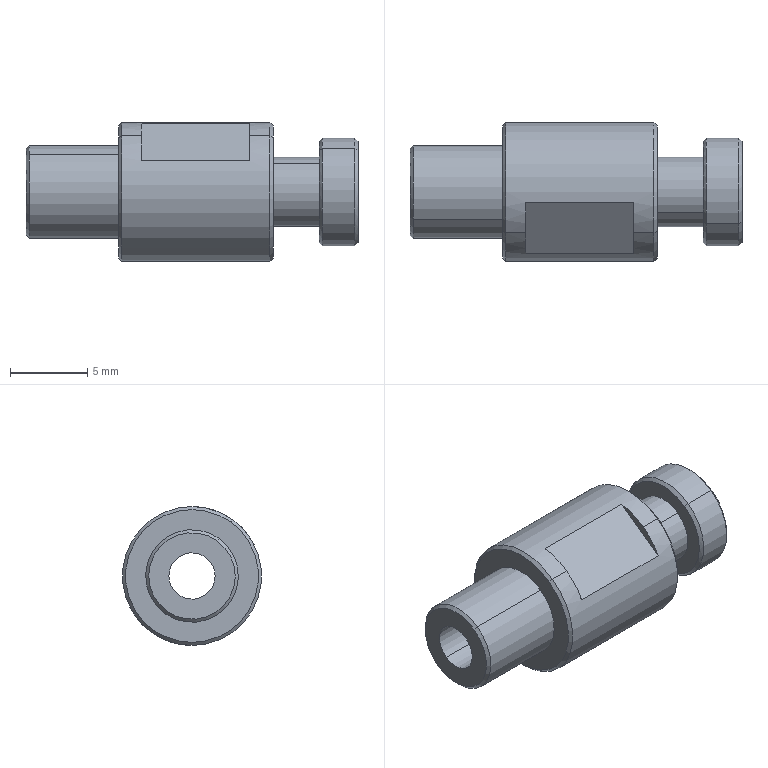Component | SolidWorks | SuctionCupConnector1-1 | 1 solid | 31 faces | box 21.5 x 9 x 9 mm | volume 776 mm3 | plane 11 | cone 10 | cylinder 10 | commonest cylinder face diameters 3 x2 6 x2 7 x2 4.5 x2 9 x2 | material 6061-T6 Aluminum
build123d program:
from build123d import *

# Parameters (mm, degrees)
SKETCH1_R           = 4.5
BOSS_EXTRUDE1_DEPTH = 5
SKETCH2_R           = 2.25
BOSS_EXTRUDE2_DEPTH = 3
SKETCH3_R           = 3.5
BOSS_EXTRUDE3_DEPTH = 2.5
SKETCH5_R           = 3
BOSS_EXTRUDE4_DEPTH = 6
SKETCH4_R           = 1.5
CUT_EXTRUDE2_DEPTH  = 23.422
CHAMFER2_SIZE       = 0.2
SKETCH6_W           = 2
SKETCH6_H           = 7
CUT_EXTRUDE3_DEPTH  = 5


with BuildPart() as part:
    # Sketch1 → Boss-Extrude1 (new, symmetric)
    with BuildSketch(Plane.XY):
        Circle(SKETCH1_R)
    extrude(amount=BOSS_EXTRUDE1_DEPTH, both=True)

    # Sketch2 → Boss-Extrude2 (add)
    with BuildSketch(Plane.XY.offset(5)):
        Circle(SKETCH2_R)
    extrude(amount=BOSS_EXTRUDE2_DEPTH)

    # Sketch3 → Boss-Extrude3 (add)
    with BuildSketch(Plane.XY.offset(8)):
        Circle(SKETCH3_R)
    extrude(amount=BOSS_EXTRUDE3_DEPTH)

    # Sketch5 → Boss-Extrude4 (add)
    with BuildSketch(Plane(origin=(0, 0, -5), x_dir=(-1, 0, 0), z_dir=(0, 0, -1))):
        with Locations(Location((0, 0, 0), (0, 0, 180))):
            Circle(SKETCH5_R)
    extrude(amount=BOSS_EXTRUDE4_DEPTH)

    # Sketch4 → Cut-Extrude2 (cut, through all)
    with BuildSketch(Plane.XY.offset(10.5)):
        Circle(SKETCH4_R)
    extrude(amount=-CUT_EXTRUDE2_DEPTH, mode=Mode.SUBTRACT)

    # Chamfer2
    chamfer2_edges = [part.edges().sort_by_distance(p)[0] for p in [
        (-3.5, 0, 8),
        (-3.5, 0, 10.5),
        (-3, 0, -11),
        (-4.5, 0, -5),
        (-4.5, 0, 5),
    ]]
    chamfer(chamfer2_edges, length=CHAMFER2_SIZE)

    # Sketch6 → Cut-Extrude3 (cut, symmetric)
    with BuildSketch(Plane(origin=(0, 0, 0), x_dir=(1, 0, 0), z_dir=(0, 1, 0))):
        with Locations((-5, 0)):
            Rectangle(SKETCH6_W, SKETCH6_H)
        with Locations((5, 0)):
            Rectangle(SKETCH6_W, SKETCH6_H)
    extrude(amount=CUT_EXTRUDE3_DEPTH, both=True, mode=Mode.SUBTRACT)


solid = part.part

# Placed as in the assembly
solid = solid.moved(Location((-566.696, -21.651, 373.468), (-144.012, 90, 0)))
STEP:
#1=CARTESIAN_POINT('',(-21.897,-0.7761,14.598));
#2=VERTEX_POINT('',#1);
#3=CARTESIAN_POINT('',(-21.897,-0.9288,14.809));
#4=VERTEX_POINT('',#3);
#5=CARTESIAN_POINT('',(-21.897,-0.8524,14.703));
#6=DIRECTION('',(1.,-0.,-0.));
#7=DIRECTION('',(0.,0.5876,-0.8091));
#8=AXIS2_PLACEMENT_3D('',#5,#6,#7);
#9=CIRCLE('',#8,0.1299);
#10=EDGE_CURVE('',#2,#4,#9,.T.);
#11=ORIENTED_EDGE('',*,*,#10,.F.);
#12=CARTESIAN_POINT('',(-21.905,-0.7714,14.592));
#13=VERTEX_POINT('',#12);
#14=CARTESIAN_POINT('',(-21.897,-0.7761,14.598));
#15=DIRECTION('',(-0.7071,0.4155,-0.5722));
#16=VECTOR('',#15,39.37);
#17=LINE('',#14,#16);
#18=EDGE_CURVE('',#2,#13,#17,.T.);
#19=ORIENTED_EDGE('',*,*,#18,.T.);
#20=CARTESIAN_POINT('',(-21.905,-0.9334,14.815));
#21=VERTEX_POINT('',#20);
#22=CARTESIAN_POINT('',(-21.905,-0.8524,14.703));
#23=DIRECTION('',(-1.,0.,0.));
#24=DIRECTION('',(0.,0.5876,-0.8091));
#25=AXIS2_PLACEMENT_3D('',#22,#23,#24);
#26=CIRCLE('',#25,0.1378);
#27=EDGE_CURVE('',#21,#13,#26,.T.);
#28=ORIENTED_EDGE('',*,*,#27,.F.);
#29=CARTESIAN_POINT('',(-21.897,-0.9288,14.809));
#30=DIRECTION('',(-0.7071,-0.4155,0.5722));
#31=VECTOR('',#30,39.37);
#32=LINE('',#29,#31);
#33=EDGE_CURVE('',#4,#21,#32,.T.);
#34=ORIENTED_EDGE('',*,*,#33,.F.);
#35=EDGE_LOOP('',(#11,#19,#28,#34));
#36=FACE_OUTER_BOUND('',#35,.T.);
#37=CARTESIAN_POINT('',(-21.897,-0.8524,14.703));
#38=DIRECTION('',(-1.,0.,0.));
#39=DIRECTION('',(0.,-0.5876,0.8091));
#40=AXIS2_PLACEMENT_3D('',#37,#38,#39);
#41=CONICAL_SURFACE('',#40,0.1299,0.7854);
#42=ADVANCED_FACE('',(#36),#41,.T.);
#43=CARTESIAN_POINT('',(-21.996,-0.9288,14.809));
#44=VERTEX_POINT('',#43);
#45=CARTESIAN_POINT('',(-21.996,-0.7761,14.598));
#46=VERTEX_POINT('',#45);
#47=CARTESIAN_POINT('',(-21.996,-0.8524,14.703));
#48=DIRECTION('',(-1.,0.,0.));
#49=DIRECTION('',(0.,0.5876,-0.8091));
#50=AXIS2_PLACEMENT_3D('',#47,#48,#49);
#51=CIRCLE('',#50,0.1299);
#52=EDGE_CURVE('',#44,#46,#51,.T.);
#53=ORIENTED_EDGE('',*,*,#52,.F.);
#54=CARTESIAN_POINT('',(-21.988,-0.9334,14.815));
#55=VERTEX_POINT('',#54);
#56=CARTESIAN_POINT('',(-21.988,-0.9334,14.815));
#57=DIRECTION('',(0.7071,-0.4155,0.5722));
#58=VECTOR('',#57,39.37);
#59=LINE('',#56,#58);
#60=EDGE_CURVE('',#44,#55,#59,.T.);
#61=ORIENTED_EDGE('',*,*,#60,.T.);
#62=CARTESIAN_POINT('',(-21.988,-0.7714,14.592));
#63=VERTEX_POINT('',#62);
#64=CARTESIAN_POINT('',(-21.988,-0.8524,14.703));
#65=DIRECTION('',(1.,-0.,-0.));
#66=DIRECTION('',(0.,0.5876,-0.8091));
#67=AXIS2_PLACEMENT_3D('',#64,#65,#66);
#68=CIRCLE('',#67,0.1378);
#69=EDGE_CURVE('',#63,#55,#68,.T.);
#70=ORIENTED_EDGE('',*,*,#69,.F.);
#71=CARTESIAN_POINT('',(-21.988,-0.7714,14.592));
#72=DIRECTION('',(0.7071,0.4155,-0.5722));
#73=VECTOR('',#72,39.37);
#74=LINE('',#71,#73);
#75=EDGE_CURVE('',#46,#63,#74,.T.);
#76=ORIENTED_EDGE('',*,*,#75,.F.);
#77=EDGE_LOOP('',(#53,#61,#70,#76));
#78=FACE_OUTER_BOUND('',#77,.T.);
#79=CARTESIAN_POINT('',(-21.988,-0.8524,14.703));
#80=DIRECTION('',(1.,-0.,-0.));
#81=DIRECTION('',(0.,0.5876,-0.8091));
#82=AXIS2_PLACEMENT_3D('',#79,#80,#81);
#83=CONICAL_SURFACE('',#82,0.1378,0.7854);
#84=ADVANCED_FACE('',(#78),#83,.T.);
#85=CARTESIAN_POINT('',(-22.114,-0.7529,14.566));
#86=VERTEX_POINT('',#85);
#87=CARTESIAN_POINT('',(-22.114,-0.9519,14.84));
#88=VERTEX_POINT('',#87);
#89=CARTESIAN_POINT('',(-22.114,-0.8524,14.703));
#90=DIRECTION('',(1.,-0.,-0.));
#91=DIRECTION('',(0.,0.5876,-0.8091));
#92=AXIS2_PLACEMENT_3D('',#89,#90,#91);
#93=CIRCLE('',#92,0.1693);
#94=EDGE_CURVE('',#86,#88,#93,.T.);
#95=ORIENTED_EDGE('',*,*,#94,.F.);
#96=CARTESIAN_POINT('',(-22.122,-0.7483,14.56));
#97=VERTEX_POINT('',#96);
#98=CARTESIAN_POINT('',(-22.114,-0.7529,14.566));
#99=DIRECTION('',(-0.7071,0.4155,-0.5722));
#100=VECTOR('',#99,39.37);
#101=LINE('',#98,#100);
#102=EDGE_CURVE('',#86,#97,#101,.T.);
#103=ORIENTED_EDGE('',*,*,#102,.T.);
#104=CARTESIAN_POINT('',(-22.122,-0.9565,14.847));
#105=VERTEX_POINT('',#104);
#106=CARTESIAN_POINT('',(-22.122,-0.8524,14.703));
#107=DIRECTION('',(-1.,0.,0.));
#108=DIRECTION('',(0.,0.5876,-0.8091));
#109=AXIS2_PLACEMENT_3D('',#106,#107,#108);
#110=CIRCLE('',#109,0.1772);
#111=EDGE_CURVE('',#105,#97,#110,.T.);
#112=ORIENTED_EDGE('',*,*,#111,.F.);
#113=CARTESIAN_POINT('',(-22.114,-0.9519,14.84));
#114=DIRECTION('',(-0.7071,-0.4155,0.5722));
#115=VECTOR('',#114,39.37);
#116=LINE('',#113,#115);
#117=EDGE_CURVE('',#88,#105,#116,.T.);
#118=ORIENTED_EDGE('',*,*,#117,.F.);
#119=EDGE_LOOP('',(#95,#103,#112,#118));
#120=FACE_OUTER_BOUND('',#119,.T.);
#121=CARTESIAN_POINT('',(-22.114,-0.8524,14.703));
#122=DIRECTION('',(-1.,0.,0.));
#123=DIRECTION('',(0.,-0.5876,0.8091));
#124=AXIS2_PLACEMENT_3D('',#121,#122,#123);
#125=CONICAL_SURFACE('',#124,0.1693,0.7854);
#126=ADVANCED_FACE('',(#120),#125,.T.);
#127=CARTESIAN_POINT('',(-22.508,-0.9519,14.84));
#128=VERTEX_POINT('',#127);
#129=CARTESIAN_POINT('',(-22.508,-0.7529,14.566));
#130=VERTEX_POINT('',#129);
#131=CARTESIAN_POINT('',(-22.508,-0.8524,14.703));
#132=DIRECTION('',(-1.,0.,0.));
#133=DIRECTION('',(0.,0.5876,-0.8091));
#134=AXIS2_PLACEMENT_3D('',#131,#132,#133);
#135=CIRCLE('',#134,0.1693);
#136=EDGE_CURVE('',#128,#130,#135,.T.);
#137=ORIENTED_EDGE('',*,*,#136,.F.);
#138=CARTESIAN_POINT('',(-22.5,-0.9565,14.847));
#139=VERTEX_POINT('',#138);
#140=CARTESIAN_POINT('',(-22.5,-0.9565,14.847));
#141=DIRECTION('',(0.7071,-0.4155,0.5722));
#142=VECTOR('',#141,39.37);
#143=LINE('',#140,#142);
#144=EDGE_CURVE('',#128,#139,#143,.T.);
#145=ORIENTED_EDGE('',*,*,#144,.T.);
#146=CARTESIAN_POINT('',(-22.5,-0.7483,14.56));
#147=VERTEX_POINT('',#146);
#148=CARTESIAN_POINT('',(-22.5,-0.8524,14.703));
#149=DIRECTION('',(1.,-0.,-0.));
#150=DIRECTION('',(0.,0.5876,-0.8091));
#151=AXIS2_PLACEMENT_3D('',#148,#149,#150);
#152=CIRCLE('',#151,0.1772);
#153=EDGE_CURVE('',#147,#139,#152,.T.);
#154=ORIENTED_EDGE('',*,*,#153,.F.);
#155=CARTESIAN_POINT('',(-22.5,-0.7483,14.56));
#156=DIRECTION('',(0.7071,0.4155,-0.5722));
#157=VECTOR('',#156,39.37);
#158=LINE('',#155,#157);
#159=EDGE_CURVE('',#130,#147,#158,.T.);
#160=ORIENTED_EDGE('',*,*,#159,.F.);
#161=EDGE_LOOP('',(#137,#145,#154,#160));
#162=FACE_OUTER_BOUND('',#161,.T.);
#163=CARTESIAN_POINT('',(-22.5,-0.8524,14.703));
#164=DIRECTION('',(1.,-0.,-0.));
#165=DIRECTION('',(0.,0.5876,-0.8091));
#166=AXIS2_PLACEMENT_3D('',#163,#164,#165);
#167=CONICAL_SURFACE('',#166,0.1772,0.7854);
#168=ADVANCED_FACE('',(#162),#167,.T.);
#169=CARTESIAN_POINT('',(-22.744,-0.9172,14.793));
#170=VERTEX_POINT('',#169);
#171=CARTESIAN_POINT('',(-22.744,-0.7876,14.614));
#172=VERTEX_POINT('',#171);
#173=CARTESIAN_POINT('',(-22.744,-0.8524,14.703));
#174=DIRECTION('',(-1.,0.,0.));
#175=DIRECTION('',(0.,-0.5876,0.8091));
#176=AXIS2_PLACEMENT_3D('',#173,#174,#175);
#177=CIRCLE('',#176,0.1102);
#178=EDGE_CURVE('',#170,#172,#177,.T.);
#179=ORIENTED_EDGE('',*,*,#178,.F.);
#180=CARTESIAN_POINT('',(-22.736,-0.9218,14.799));
#181=VERTEX_POINT('',#180);
#182=CARTESIAN_POINT('',(-22.744,-0.9172,14.793));
#183=DIRECTION('',(0.7071,-0.4155,0.5722));
#184=VECTOR('',#183,39.37);
#185=LINE('',#182,#184);
#186=EDGE_CURVE('',#170,#181,#185,.T.);
#187=ORIENTED_EDGE('',*,*,#186,.T.);
#188=CARTESIAN_POINT('',(-22.736,-0.783,14.608));
#189=VERTEX_POINT('',#188);
#190=CARTESIAN_POINT('',(-22.736,-0.8524,14.703));
#191=DIRECTION('',(1.,-0.,-0.));
#192=DIRECTION('',(0.,-0.5876,0.8091));
#193=AXIS2_PLACEMENT_3D('',#190,#191,#192);
#194=CIRCLE('',#193,0.1181);
#195=EDGE_CURVE('',#189,#181,#194,.T.);
#196=ORIENTED_EDGE('',*,*,#195,.F.);
#197=CARTESIAN_POINT('',(-22.744,-0.7876,14.614));
#198=DIRECTION('',(0.7071,0.4155,-0.5722));
#199=VECTOR('',#198,39.37);
#200=LINE('',#197,#199);
#201=EDGE_CURVE('',#172,#189,#200,.T.);
#202=ORIENTED_EDGE('',*,*,#201,.F.);
#203=EDGE_LOOP('',(#179,#187,#196,#202));
#204=FACE_OUTER_BOUND('',#203,.T.);
#205=CARTESIAN_POINT('',(-22.744,-0.8524,14.703));
#206=DIRECTION('',(1.,-0.,-0.));
#207=DIRECTION('',(0.,0.5876,-0.8091));
#208=AXIS2_PLACEMENT_3D('',#205,#206,#207);
#209=CONICAL_SURFACE('',#208,0.1102,0.7854);
#210=ADVANCED_FACE('',(#204),#209,.T.);
#211=CARTESIAN_POINT('',(-22.744,-0.8871,14.751));
#212=VERTEX_POINT('',#211);
#213=CARTESIAN_POINT('',(-22.744,-0.8177,14.656));
#214=VERTEX_POINT('',#213);
#215=CARTESIAN_POINT('',(-22.744,-0.8524,14.703));
#216=DIRECTION('',(1.,-0.,-0.));
#217=DIRECTION('',(0.,0.5876,-0.8091));
#218=AXIS2_PLACEMENT_3D('',#215,#216,#217);
#219=CIRCLE('',#218,0.05906);
#220=EDGE_CURVE('',#212,#214,#219,.T.);
#221=ORIENTED_EDGE('',*,*,#220,.F.);
#222=CARTESIAN_POINT('',(-21.897,-0.8871,14.751));
#223=VERTEX_POINT('',#222);
#224=CARTESIAN_POINT('',(-22.744,-0.8871,14.751));
#225=DIRECTION('',(1.,-0.,-0.));
#226=VECTOR('',#225,39.37);
#227=LINE('',#224,#226);
#228=EDGE_CURVE('',#212,#223,#227,.T.);
#229=ORIENTED_EDGE('',*,*,#228,.T.);
#230=CARTESIAN_POINT('',(-21.897,-0.8177,14.656));
#231=VERTEX_POINT('',#230);
#232=CARTESIAN_POINT('',(-21.897,-0.8524,14.703));
#233=DIRECTION('',(1.,-0.,-0.));
#234=DIRECTION('',(0.,0.5876,-0.8091));
#235=AXIS2_PLACEMENT_3D('',#232,#233,#234);
#236=CIRCLE('',#235,0.05906);
#237=EDGE_CURVE('',#223,#231,#236,.T.);
#238=ORIENTED_EDGE('',*,*,#237,.T.);
#239=CARTESIAN_POINT('',(-22.744,-0.8177,14.656));
#240=DIRECTION('',(1.,-0.,-0.));
#241=VECTOR('',#240,39.37);
#242=LINE('',#239,#241);
#243=EDGE_CURVE('',#214,#231,#242,.T.);
#244=ORIENTED_EDGE('',*,*,#243,.F.);
#245=EDGE_LOOP('',(#221,#229,#238,#244));
#246=FACE_OUTER_BOUND('',#245,.T.);
#247=CARTESIAN_POINT('',(-22.744,-0.8524,14.703));
#248=DIRECTION('',(1.,-0.,-0.));
#249=DIRECTION('',(0.,0.5876,-0.8091));
#250=AXIS2_PLACEMENT_3D('',#247,#248,#249);
#251=CYLINDRICAL_SURFACE('',#250,0.05906);
#252=ADVANCED_FACE('',(#246),#251,.F.);
#253=ORIENTED_EDGE('',*,*,#195,.T.);
#254=CARTESIAN_POINT('',(-22.508,-0.9218,14.799));
#255=VERTEX_POINT('',#254);
#256=CARTESIAN_POINT('',(-22.744,-0.9218,14.799));
#257=DIRECTION('',(1.,-0.,-0.));
#258=VECTOR('',#257,39.37);
#259=LINE('',#256,#258);
#260=EDGE_CURVE('',#181,#255,#259,.T.);
#261=ORIENTED_EDGE('',*,*,#260,.T.);
#262=CARTESIAN_POINT('',(-22.508,-0.783,14.608));
#263=VERTEX_POINT('',#262);
#264=CARTESIAN_POINT('',(-22.508,-0.8524,14.703));
#265=DIRECTION('',(-1.,0.,0.));
#266=DIRECTION('',(0.,0.5876,-0.8091));
#267=AXIS2_PLACEMENT_3D('',#264,#265,#266);
#268=CIRCLE('',#267,0.1181);
#269=EDGE_CURVE('',#255,#263,#268,.T.);
#270=ORIENTED_EDGE('',*,*,#269,.T.);
#271=CARTESIAN_POINT('',(-22.744,-0.783,14.608));
#272=DIRECTION('',(1.,-0.,-0.));
#273=VECTOR('',#272,39.37);
#274=LINE('',#271,#273);
#275=EDGE_CURVE('',#189,#263,#274,.T.);
#276=ORIENTED_EDGE('',*,*,#275,.F.);
#277=EDGE_LOOP('',(#253,#261,#270,#276));
#278=FACE_OUTER_BOUND('',#277,.T.);
#279=CARTESIAN_POINT('',(-22.744,-0.8524,14.703));
#280=DIRECTION('',(1.,-0.,-0.));
#281=DIRECTION('',(0.,0.5876,-0.8091));
#282=AXIS2_PLACEMENT_3D('',#279,#280,#281);
#283=CYLINDRICAL_SURFACE('',#282,0.1181);
#284=ADVANCED_FACE('',(#278),#283,.T.);
#285=ORIENTED_EDGE('',*,*,#27,.T.);
#286=CARTESIAN_POINT('',(-21.897,-0.7714,14.592));
#287=DIRECTION('',(-1.,0.,0.));
#288=VECTOR('',#287,39.37);
#289=LINE('',#286,#288);
#290=EDGE_CURVE('',#13,#63,#289,.T.);
#291=ORIENTED_EDGE('',*,*,#290,.T.);
#292=ORIENTED_EDGE('',*,*,#69,.T.);
#293=CARTESIAN_POINT('',(-21.897,-0.9334,14.815));
#294=DIRECTION('',(-1.,0.,0.));
#295=VECTOR('',#294,39.37);
#296=LINE('',#293,#295);
#297=EDGE_CURVE('',#21,#55,#296,.T.);
#298=ORIENTED_EDGE('',*,*,#297,.F.);
#299=EDGE_LOOP('',(#285,#291,#292,#298));
#300=FACE_OUTER_BOUND('',#299,.T.);
#301=CARTESIAN_POINT('',(-21.897,-0.8524,14.703));
#302=DIRECTION('',(-1.,0.,0.));
#303=DIRECTION('',(0.,-0.5876,0.8091));
#304=AXIS2_PLACEMENT_3D('',#301,#302,#303);
#305=CYLINDRICAL_SURFACE('',#304,0.1378);
#306=ADVANCED_FACE('',(#300),#305,.T.);
#307=CARTESIAN_POINT('',(-21.996,-0.8004,14.632));
#308=VERTEX_POINT('',#307);
#309=CARTESIAN_POINT('',(-21.996,-0.9045,14.775));
#310=VERTEX_POINT('',#309);
#311=CARTESIAN_POINT('',(-21.996,-0.8524,14.703));
#312=DIRECTION('',(1.,-0.,-0.));
#313=DIRECTION('',(0.,0.5876,-0.8091));
#314=AXIS2_PLACEMENT_3D('',#311,#312,#313);
#315=CIRCLE('',#314,0.08858);
#316=EDGE_CURVE('',#308,#310,#315,.T.);
#317=ORIENTED_EDGE('',*,*,#316,.F.);
#318=CARTESIAN_POINT('',(-22.114,-0.8004,14.632));
#319=VERTEX_POINT('',#318);
#320=CARTESIAN_POINT('',(-21.996,-0.8004,14.632));
#321=DIRECTION('',(-1.,0.,0.));
#322=VECTOR('',#321,39.37);
#323=LINE('',#320,#322);
#324=EDGE_CURVE('',#308,#319,#323,.T.);
#325=ORIENTED_EDGE('',*,*,#324,.T.);
#326=CARTESIAN_POINT('',(-22.114,-0.9045,14.775));
#327=VERTEX_POINT('',#326);
#328=CARTESIAN_POINT('',(-22.114,-0.8524,14.703));
#329=DIRECTION('',(1.,-0.,-0.));
#330=DIRECTION('',(0.,0.5876,-0.8091));
#331=AXIS2_PLACEMENT_3D('',#328,#329,#330);
#332=CIRCLE('',#331,0.08858);
#333=EDGE_CURVE('',#319,#327,#332,.T.);
#334=ORIENTED_EDGE('',*,*,#333,.T.);
#335=CARTESIAN_POINT('',(-21.996,-0.9045,14.775));
#336=DIRECTION('',(-1.,0.,0.));
#337=VECTOR('',#336,39.37);
#338=LINE('',#335,#337);
#339=EDGE_CURVE('',#310,#327,#338,.T.);
#340=ORIENTED_EDGE('',*,*,#339,.F.);
#341=EDGE_LOOP('',(#317,#325,#334,#340));
#342=FACE_OUTER_BOUND('',#341,.T.);
#343=CARTESIAN_POINT('',(-21.996,-0.8524,14.703));
#344=DIRECTION('',(-1.,0.,0.));
#345=DIRECTION('',(0.,-0.5876,0.8091));
#346=AXIS2_PLACEMENT_3D('',#343,#344,#345);
#347=CYLINDRICAL_SURFACE('',#346,0.08858);
#348=ADVANCED_FACE('',(#342),#347,.T.);
#349=ORIENTED_EDGE('',*,*,#111,.T.);
#350=CARTESIAN_POINT('',(-22.173,-0.7483,14.56));
#351=VERTEX_POINT('',#350);
#352=CARTESIAN_POINT('',(-22.114,-0.7483,14.56));
#353=DIRECTION('',(-1.,0.,0.));
#354=VECTOR('',#353,39.37);
#355=LINE('',#352,#354);
#356=EDGE_CURVE('',#97,#351,#355,.T.);
#357=ORIENTED_EDGE('',*,*,#356,.T.);
#358=CARTESIAN_POINT('',(-22.173,-0.6942,14.624));
#359=VERTEX_POINT('',#358);
#360=CARTESIAN_POINT('',(-22.173,-0.8524,14.703));
#361=DIRECTION('',(1.,-0.,0.));
#362=DIRECTION('',(0.,0.5876,-0.8091));
#363=AXIS2_PLACEMENT_3D('',#360,#361,#362);
#364=CIRCLE('',#363,0.1772);
#365=EDGE_CURVE('',#351,#359,#364,.T.);
#366=ORIENTED_EDGE('',*,*,#365,.T.);
#367=CARTESIAN_POINT('',(-22.449,-0.6942,14.624));
#368=VERTEX_POINT('',#367);
#369=CARTESIAN_POINT('',(-22.114,-0.6942,14.624));
#370=DIRECTION('',(-1.,0.,0.));
#371=VECTOR('',#370,39.37);
#372=LINE('',#369,#371);
#373=EDGE_CURVE('',#359,#368,#372,.T.);
#374=ORIENTED_EDGE('',*,*,#373,.T.);
#375=CARTESIAN_POINT('',(-22.449,-0.7483,14.56));
#376=VERTEX_POINT('',#375);
#377=CARTESIAN_POINT('',(-22.449,-0.8524,14.703));
#378=DIRECTION('',(-1.,-0.,0.));
#379=DIRECTION('',(0.,-0.5876,0.8091));
#380=AXIS2_PLACEMENT_3D('',#377,#378,#379);
#381=CIRCLE('',#380,0.1772);
#382=EDGE_CURVE('',#368,#376,#381,.T.);
#383=ORIENTED_EDGE('',*,*,#382,.T.);
#384=CARTESIAN_POINT('',(-22.114,-0.7483,14.56));
#385=DIRECTION('',(-1.,0.,0.));
#386=VECTOR('',#385,39.37);
#387=LINE('',#384,#386);
#388=EDGE_CURVE('',#376,#147,#387,.T.);
#389=ORIENTED_EDGE('',*,*,#388,.T.);
#390=ORIENTED_EDGE('',*,*,#153,.T.);
#391=CARTESIAN_POINT('',(-22.449,-0.9565,14.847));
#392=VERTEX_POINT('',#391);
#393=CARTESIAN_POINT('',(-22.114,-0.9565,14.847));
#394=DIRECTION('',(-1.,0.,0.));
#395=VECTOR('',#394,39.37);
#396=LINE('',#393,#395);
#397=EDGE_CURVE('',#392,#139,#396,.T.);
#398=ORIENTED_EDGE('',*,*,#397,.F.);
#399=CARTESIAN_POINT('',(-22.449,-0.8793,14.879));
#400=VERTEX_POINT('',#399);
#401=CARTESIAN_POINT('',(-22.449,-0.8524,14.703));
#402=DIRECTION('',(-1.,0.,0.));
#403=DIRECTION('',(0.,-0.5876,0.8091));
#404=AXIS2_PLACEMENT_3D('',#401,#402,#403);
#405=CIRCLE('',#404,0.1772);
#406=EDGE_CURVE('',#392,#400,#405,.T.);
#407=ORIENTED_EDGE('',*,*,#406,.T.);
#408=CARTESIAN_POINT('',(-22.173,-0.8793,14.879));
#409=VERTEX_POINT('',#408);
#410=CARTESIAN_POINT('',(-22.114,-0.8793,14.879));
#411=DIRECTION('',(1.,-0.,-0.));
#412=VECTOR('',#411,39.37);
#413=LINE('',#410,#412);
#414=EDGE_CURVE('',#400,#409,#413,.T.);
#415=ORIENTED_EDGE('',*,*,#414,.T.);
#416=CARTESIAN_POINT('',(-22.173,-0.9565,14.847));
#417=VERTEX_POINT('',#416);
#418=CARTESIAN_POINT('',(-22.173,-0.8524,14.703));
#419=DIRECTION('',(1.,0.,-0.));
#420=DIRECTION('',(0.,0.5876,-0.8091));
#421=AXIS2_PLACEMENT_3D('',#418,#419,#420);
#422=CIRCLE('',#421,0.1772);
#423=EDGE_CURVE('',#409,#417,#422,.T.);
#424=ORIENTED_EDGE('',*,*,#423,.T.);
#425=CARTESIAN_POINT('',(-22.114,-0.9565,14.847));
#426=DIRECTION('',(-1.,0.,0.));
#427=VECTOR('',#426,39.37);
#428=LINE('',#425,#427);
#429=EDGE_CURVE('',#105,#417,#428,.T.);
#430=ORIENTED_EDGE('',*,*,#429,.F.);
#431=EDGE_LOOP('',(#349,#357,#366,#374,#383,#389,#390,#398,#407,#415,#424,#430));
#432=FACE_OUTER_BOUND('',#431,.T.);
#433=CARTESIAN_POINT('',(-22.114,-0.8524,14.703));
#434=DIRECTION('',(-1.,0.,0.));
#435=DIRECTION('',(0.,-0.5876,0.8091));
#436=AXIS2_PLACEMENT_3D('',#433,#434,#435);
#437=CYLINDRICAL_SURFACE('',#436,0.1772);
#438=ADVANCED_FACE('',(#432),#437,.T.);
#439=CARTESIAN_POINT('',(-22.508,-0.8524,14.703));
#440=DIRECTION('',(-1.,0.,0.));
#441=DIRECTION('',(0.,0.5876,-0.8091));
#442=AXIS2_PLACEMENT_3D('',#439,#440,#441);
#443=CIRCLE('',#442,0.1693);
#444=EDGE_CURVE('',#130,#128,#443,.T.);
#445=ORIENTED_EDGE('',*,*,#444,.T.);
#446=ORIENTED_EDGE('',*,*,#136,.T.);
#447=EDGE_LOOP('',(#445,#446));
#448=FACE_OUTER_BOUND('',#447,.T.);
#449=CARTESIAN_POINT('',(-22.508,-0.8524,14.703));
#450=DIRECTION('',(-1.,0.,0.));
#451=DIRECTION('',(0.,0.5876,-0.8091));
#452=AXIS2_PLACEMENT_3D('',#449,#450,#451);
#453=CIRCLE('',#452,0.1181);
#454=EDGE_CURVE('',#263,#255,#453,.T.);
#455=ORIENTED_EDGE('',*,*,#454,.F.);
#456=ORIENTED_EDGE('',*,*,#269,.F.);
#457=EDGE_LOOP('',(#455,#456));
#458=FACE_BOUND('',#457,.T.);
#459=CARTESIAN_POINT('',(-22.508,-0.8524,14.703));
#460=DIRECTION('',(1.,-0.,-0.));
#461=DIRECTION('',(-0.,0.5876,-0.8091));
#462=AXIS2_PLACEMENT_3D('',#459,#460,#461);
#463=PLANE('',#462);
#464=ADVANCED_FACE('',(#448,#458),#463,.F.);
#465=CARTESIAN_POINT('',(-22.114,-0.8524,14.703));
#466=DIRECTION('',(1.,-0.,-0.));
#467=DIRECTION('',(0.,0.5876,-0.8091));
#468=AXIS2_PLACEMENT_3D('',#465,#466,#467);
#469=CIRCLE('',#468,0.1693);
#470=EDGE_CURVE('',#88,#86,#469,.T.);
#471=ORIENTED_EDGE('',*,*,#470,.T.);
#472=ORIENTED_EDGE('',*,*,#94,.T.);
#473=EDGE_LOOP('',(#471,#472));
#474=FACE_OUTER_BOUND('',#473,.T.);
#475=CARTESIAN_POINT('',(-22.114,-0.8524,14.703));
#476=DIRECTION('',(1.,-0.,-0.));
#477=DIRECTION('',(0.,0.5876,-0.8091));
#478=AXIS2_PLACEMENT_3D('',#475,#476,#477);
#479=CIRCLE('',#478,0.08858);
#480=EDGE_CURVE('',#327,#319,#479,.T.);
#481=ORIENTED_EDGE('',*,*,#480,.F.);
#482=ORIENTED_EDGE('',*,*,#333,.F.);
#483=EDGE_LOOP('',(#481,#482));
#484=FACE_BOUND('',#483,.T.);
#485=CARTESIAN_POINT('',(-22.114,-0.8524,14.703));
#486=DIRECTION('',(1.,-0.,-0.));
#487=DIRECTION('',(-0.,0.5876,-0.8091));
#488=AXIS2_PLACEMENT_3D('',#485,#486,#487);
#489=PLANE('',#488);
#490=ADVANCED_FACE('',(#474,#484),#489,.T.);
#491=ORIENTED_EDGE('',*,*,#356,.F.);
#492=CARTESIAN_POINT('',(-22.122,-0.8524,14.703));
#493=DIRECTION('',(-1.,0.,0.));
#494=DIRECTION('',(0.,0.5876,-0.8091));
#495=AXIS2_PLACEMENT_3D('',#492,#493,#494);
#496=CIRCLE('',#495,0.1772);
#497=EDGE_CURVE('',#97,#105,#496,.T.);
#498=ORIENTED_EDGE('',*,*,#497,.T.);
#499=ORIENTED_EDGE('',*,*,#429,.T.);
#500=CARTESIAN_POINT('',(-22.173,-1.011,14.783));
#501=VERTEX_POINT('',#500);
#502=CARTESIAN_POINT('',(-22.173,-0.8524,14.703));
#503=DIRECTION('',(1.,0.,-0.));
#504=DIRECTION('',(0.,0.5876,-0.8091));
#505=AXIS2_PLACEMENT_3D('',#502,#503,#504);
#506=CIRCLE('',#505,0.1772);
#507=EDGE_CURVE('',#417,#501,#506,.T.);
#508=ORIENTED_EDGE('',*,*,#507,.T.);
#509=CARTESIAN_POINT('',(-22.449,-1.011,14.783));
#510=VERTEX_POINT('',#509);
#511=CARTESIAN_POINT('',(-22.114,-1.011,14.783));
#512=DIRECTION('',(-1.,0.,0.));
#513=VECTOR('',#512,39.37);
#514=LINE('',#511,#513);
#515=EDGE_CURVE('',#501,#510,#514,.T.);
#516=ORIENTED_EDGE('',*,*,#515,.T.);
#517=CARTESIAN_POINT('',(-22.449,-0.8524,14.703));
#518=DIRECTION('',(-1.,0.,0.));
#519=DIRECTION('',(0.,-0.5876,0.8091));
#520=AXIS2_PLACEMENT_3D('',#517,#518,#519);
#521=CIRCLE('',#520,0.1772);
#522=EDGE_CURVE('',#510,#392,#521,.T.);
#523=ORIENTED_EDGE('',*,*,#522,.T.);
#524=ORIENTED_EDGE('',*,*,#397,.T.);
#525=CARTESIAN_POINT('',(-22.5,-0.8524,14.703));
#526=DIRECTION('',(1.,-0.,-0.));
#527=DIRECTION('',(0.,0.5876,-0.8091));
#528=AXIS2_PLACEMENT_3D('',#525,#526,#527);
#529=CIRCLE('',#528,0.1772);
#530=EDGE_CURVE('',#139,#147,#529,.T.);
#531=ORIENTED_EDGE('',*,*,#530,.T.);
#532=ORIENTED_EDGE('',*,*,#388,.F.);
#533=CARTESIAN_POINT('',(-22.449,-0.8256,14.528));
#534=VERTEX_POINT('',#533);
#535=CARTESIAN_POINT('',(-22.449,-0.8524,14.703));
#536=DIRECTION('',(-1.,-0.,0.));
#537=DIRECTION('',(0.,-0.5876,0.8091));
#538=AXIS2_PLACEMENT_3D('',#535,#536,#537);
#539=CIRCLE('',#538,0.1772);
#540=EDGE_CURVE('',#376,#534,#539,.T.);
#541=ORIENTED_EDGE('',*,*,#540,.T.);
#542=CARTESIAN_POINT('',(-22.173,-0.8256,14.528));
#543=VERTEX_POINT('',#542);
#544=CARTESIAN_POINT('',(-22.114,-0.8256,14.528));
#545=DIRECTION('',(1.,-0.,-0.));
#546=VECTOR('',#545,39.37);
#547=LINE('',#544,#546);
#548=EDGE_CURVE('',#534,#543,#547,.T.);
#549=ORIENTED_EDGE('',*,*,#548,.T.);
#550=CARTESIAN_POINT('',(-22.173,-0.8524,14.703));
#551=DIRECTION('',(1.,-0.,0.));
#552=DIRECTION('',(0.,0.5876,-0.8091));
#553=AXIS2_PLACEMENT_3D('',#550,#551,#552);
#554=CIRCLE('',#553,0.1772);
#555=EDGE_CURVE('',#543,#351,#554,.T.);
#556=ORIENTED_EDGE('',*,*,#555,.T.);
#557=EDGE_LOOP('',(#491,#498,#499,#508,#516,#523,#524,#531,#532,#541,#549,#556));
#558=FACE_OUTER_BOUND('',#557,.T.);
#559=CARTESIAN_POINT('',(-22.114,-0.8524,14.703));
#560=DIRECTION('',(-1.,0.,0.));
#561=DIRECTION('',(0.,-0.5876,0.8091));
#562=AXIS2_PLACEMENT_3D('',#559,#560,#561);
#563=CYLINDRICAL_SURFACE('',#562,0.1772);
#564=ADVANCED_FACE('',(#558),#563,.T.);
#565=ORIENTED_EDGE('',*,*,#324,.F.);
#566=CARTESIAN_POINT('',(-21.996,-0.8524,14.703));
#567=DIRECTION('',(1.,-0.,-0.));
#568=DIRECTION('',(0.,0.5876,-0.8091));
#569=AXIS2_PLACEMENT_3D('',#566,#567,#568);
#570=CIRCLE('',#569,0.08858);
#571=EDGE_CURVE('',#310,#308,#570,.T.);
#572=ORIENTED_EDGE('',*,*,#571,.F.);
#573=ORIENTED_EDGE('',*,*,#339,.T.);
#574=ORIENTED_EDGE('',*,*,#480,.T.);
#575=EDGE_LOOP('',(#565,#572,#573,#574));
#576=FACE_OUTER_BOUND('',#575,.T.);
#577=CARTESIAN_POINT('',(-21.996,-0.8524,14.703));
#578=DIRECTION('',(-1.,0.,0.));
#579=DIRECTION('',(0.,-0.5876,0.8091));
#580=AXIS2_PLACEMENT_3D('',#577,#578,#579);
#581=CYLINDRICAL_SURFACE('',#580,0.08858);
#582=ADVANCED_FACE('',(#576),#581,.T.);
#583=CARTESIAN_POINT('',(-21.996,-0.8524,14.703));
#584=DIRECTION('',(-1.,0.,0.));
#585=DIRECTION('',(0.,0.5876,-0.8091));
#586=AXIS2_PLACEMENT_3D('',#583,#584,#585);
#587=CIRCLE('',#586,0.1299);
#588=EDGE_CURVE('',#46,#44,#587,.T.);
#589=ORIENTED_EDGE('',*,*,#588,.T.);
#590=ORIENTED_EDGE('',*,*,#52,.T.);
#591=EDGE_LOOP('',(#589,#590));
#592=FACE_OUTER_BOUND('',#591,.T.);
#593=ORIENTED_EDGE('',*,*,#571,.T.);
#594=ORIENTED_EDGE('',*,*,#316,.T.);
#595=EDGE_LOOP('',(#593,#594));
#596=FACE_BOUND('',#595,.T.);
#597=CARTESIAN_POINT('',(-21.996,-0.8524,14.703));
#598=DIRECTION('',(1.,-0.,-0.));
#599=DIRECTION('',(-0.,0.5876,-0.8091));
#600=AXIS2_PLACEMENT_3D('',#597,#598,#599);
#601=PLANE('',#600);
#602=ADVANCED_FACE('',(#592,#596),#601,.F.);
#603=ORIENTED_EDGE('',*,*,#290,.F.);
#604=CARTESIAN_POINT('',(-21.905,-0.8524,14.703));
#605=DIRECTION('',(-1.,0.,0.));
#606=DIRECTION('',(0.,0.5876,-0.8091));
#607=AXIS2_PLACEMENT_3D('',#604,#605,#606);
#608=CIRCLE('',#607,0.1378);
#609=EDGE_CURVE('',#13,#21,#608,.T.);
#610=ORIENTED_EDGE('',*,*,#609,.T.);
#611=ORIENTED_EDGE('',*,*,#297,.T.);
#612=CARTESIAN_POINT('',(-21.988,-0.8524,14.703));
#613=DIRECTION('',(1.,-0.,-0.));
#614=DIRECTION('',(0.,0.5876,-0.8091));
#615=AXIS2_PLACEMENT_3D('',#612,#613,#614);
#616=CIRCLE('',#615,0.1378);
#617=EDGE_CURVE('',#55,#63,#616,.T.);
#618=ORIENTED_EDGE('',*,*,#617,.T.);
#619=EDGE_LOOP('',(#603,#610,#611,#618));
#620=FACE_OUTER_BOUND('',#619,.T.);
#621=CARTESIAN_POINT('',(-21.897,-0.8524,14.703));
#622=DIRECTION('',(-1.,0.,0.));
#623=DIRECTION('',(0.,-0.5876,0.8091));
#624=AXIS2_PLACEMENT_3D('',#621,#622,#623);
#625=CYLINDRICAL_SURFACE('',#624,0.1378);
#626=ADVANCED_FACE('',(#620),#625,.T.);
#627=CARTESIAN_POINT('',(-21.897,-0.8524,14.703));
#628=DIRECTION('',(1.,-0.,-0.));
#629=DIRECTION('',(0.,0.5876,-0.8091));
#630=AXIS2_PLACEMENT_3D('',#627,#628,#629);
#631=CIRCLE('',#630,0.1299);
#632=EDGE_CURVE('',#4,#2,#631,.T.);
#633=ORIENTED_EDGE('',*,*,#632,.T.);
#634=ORIENTED_EDGE('',*,*,#10,.T.);
#635=EDGE_LOOP('',(#633,#634));
#636=FACE_OUTER_BOUND('',#635,.T.);
#637=CARTESIAN_POINT('',(-21.897,-0.8524,14.703));
#638=DIRECTION('',(1.,-0.,-0.));
#639=DIRECTION('',(0.,0.5876,-0.8091));
#640=AXIS2_PLACEMENT_3D('',#637,#638,#639);
#641=CIRCLE('',#640,0.05906);
#642=EDGE_CURVE('',#231,#223,#641,.T.);
#643=ORIENTED_EDGE('',*,*,#642,.F.);
#644=ORIENTED_EDGE('',*,*,#237,.F.);
#645=EDGE_LOOP('',(#643,#644));
#646=FACE_BOUND('',#645,.T.);
#647=CARTESIAN_POINT('',(-21.897,-0.8524,14.703));
#648=DIRECTION('',(1.,-0.,-0.));
#649=DIRECTION('',(-0.,0.5876,-0.8091));
#650=AXIS2_PLACEMENT_3D('',#647,#648,#649);
#651=PLANE('',#650);
#652=ADVANCED_FACE('',(#636,#646),#651,.T.);
#653=ORIENTED_EDGE('',*,*,#260,.F.);
#654=CARTESIAN_POINT('',(-22.736,-0.8524,14.703));
#655=DIRECTION('',(1.,-0.,-0.));
#656=DIRECTION('',(0.,-0.5876,0.8091));
#657=AXIS2_PLACEMENT_3D('',#654,#655,#656);
#658=CIRCLE('',#657,0.1181);
#659=EDGE_CURVE('',#181,#189,#658,.T.);
#660=ORIENTED_EDGE('',*,*,#659,.T.);
#661=ORIENTED_EDGE('',*,*,#275,.T.);
#662=ORIENTED_EDGE('',*,*,#454,.T.);
#663=EDGE_LOOP('',(#653,#660,#661,#662));
#664=FACE_OUTER_BOUND('',#663,.T.);
#665=CARTESIAN_POINT('',(-22.744,-0.8524,14.703));
#666=DIRECTION('',(1.,-0.,-0.));
#667=DIRECTION('',(0.,0.5876,-0.8091));
#668=AXIS2_PLACEMENT_3D('',#665,#666,#667);
#669=CYLINDRICAL_SURFACE('',#668,0.1181);
#670=ADVANCED_FACE('',(#664),#669,.T.);
#671=CARTESIAN_POINT('',(-22.744,-0.8524,14.703));
#672=DIRECTION('',(-1.,0.,0.));
#673=DIRECTION('',(0.,-0.5876,0.8091));
#674=AXIS2_PLACEMENT_3D('',#671,#672,#673);
#675=CIRCLE('',#674,0.1102);
#676=EDGE_CURVE('',#172,#170,#675,.T.);
#677=ORIENTED_EDGE('',*,*,#676,.T.);
#678=ORIENTED_EDGE('',*,*,#178,.T.);
#679=EDGE_LOOP('',(#677,#678));
#680=FACE_OUTER_BOUND('',#679,.T.);
#681=CARTESIAN_POINT('',(-22.744,-0.8524,14.703));
#682=DIRECTION('',(1.,-0.,-0.));
#683=DIRECTION('',(0.,0.5876,-0.8091));
#684=AXIS2_PLACEMENT_3D('',#681,#682,#683);
#685=CIRCLE('',#684,0.05906);
#686=EDGE_CURVE('',#214,#212,#685,.T.);
#687=ORIENTED_EDGE('',*,*,#686,.T.);
#688=ORIENTED_EDGE('',*,*,#220,.T.);
#689=EDGE_LOOP('',(#687,#688));
#690=FACE_BOUND('',#689,.T.);
#691=CARTESIAN_POINT('',(-22.744,-0.8524,14.703));
#692=DIRECTION('',(-1.,0.,0.));
#693=DIRECTION('',(0.,-0.5876,0.8091));
#694=AXIS2_PLACEMENT_3D('',#691,#692,#693);
#695=PLANE('',#694);
#696=ADVANCED_FACE('',(#680,#690),#695,.T.);
#697=ORIENTED_EDGE('',*,*,#228,.F.);
#698=ORIENTED_EDGE('',*,*,#686,.F.);
#699=ORIENTED_EDGE('',*,*,#243,.T.);
#700=ORIENTED_EDGE('',*,*,#642,.T.);
#701=EDGE_LOOP('',(#697,#698,#699,#700));
#702=FACE_OUTER_BOUND('',#701,.T.);
#703=CARTESIAN_POINT('',(-22.744,-0.8524,14.703));
#704=DIRECTION('',(1.,-0.,-0.));
#705=DIRECTION('',(0.,0.5876,-0.8091));
#706=AXIS2_PLACEMENT_3D('',#703,#704,#705);
#707=CYLINDRICAL_SURFACE('',#706,0.05906);
#708=ADVANCED_FACE('',(#702),#707,.F.);
#709=ORIENTED_EDGE('',*,*,#186,.F.);
#710=ORIENTED_EDGE('',*,*,#676,.F.);
#711=ORIENTED_EDGE('',*,*,#201,.T.);
#712=ORIENTED_EDGE('',*,*,#659,.F.);
#713=EDGE_LOOP('',(#709,#710,#711,#712));
#714=FACE_OUTER_BOUND('',#713,.T.);
#715=CARTESIAN_POINT('',(-22.744,-0.8524,14.703));
#716=DIRECTION('',(1.,-0.,-0.));
#717=DIRECTION('',(0.,0.5876,-0.8091));
#718=AXIS2_PLACEMENT_3D('',#715,#716,#717);
#719=CONICAL_SURFACE('',#718,0.1102,0.7854);
#720=ADVANCED_FACE('',(#714),#719,.T.);
#721=ORIENTED_EDGE('',*,*,#144,.F.);
#722=ORIENTED_EDGE('',*,*,#444,.F.);
#723=ORIENTED_EDGE('',*,*,#159,.T.);
#724=ORIENTED_EDGE('',*,*,#530,.F.);
#725=EDGE_LOOP('',(#721,#722,#723,#724));
#726=FACE_OUTER_BOUND('',#725,.T.);
#727=CARTESIAN_POINT('',(-22.5,-0.8524,14.703));
#728=DIRECTION('',(1.,-0.,-0.));
#729=DIRECTION('',(0.,0.5876,-0.8091));
#730=AXIS2_PLACEMENT_3D('',#727,#728,#729);
#731=CONICAL_SURFACE('',#730,0.1772,0.7854);
#732=ADVANCED_FACE('',(#726),#731,.T.);
#733=ORIENTED_EDGE('',*,*,#102,.F.);
#734=ORIENTED_EDGE('',*,*,#470,.F.);
#735=ORIENTED_EDGE('',*,*,#117,.T.);
#736=ORIENTED_EDGE('',*,*,#497,.F.);
#737=EDGE_LOOP('',(#733,#734,#735,#736));
#738=FACE_OUTER_BOUND('',#737,.T.);
#739=CARTESIAN_POINT('',(-22.114,-0.8524,14.703));
#740=DIRECTION('',(-1.,0.,0.));
#741=DIRECTION('',(0.,-0.5876,0.8091));
#742=AXIS2_PLACEMENT_3D('',#739,#740,#741);
#743=CONICAL_SURFACE('',#742,0.1693,0.7854);
#744=ADVANCED_FACE('',(#738),#743,.T.);
#745=ORIENTED_EDGE('',*,*,#60,.F.);
#746=ORIENTED_EDGE('',*,*,#588,.F.);
#747=ORIENTED_EDGE('',*,*,#75,.T.);
#748=ORIENTED_EDGE('',*,*,#617,.F.);
#749=EDGE_LOOP('',(#745,#746,#747,#748));
#750=FACE_OUTER_BOUND('',#749,.T.);
#751=CARTESIAN_POINT('',(-21.988,-0.8524,14.703));
#752=DIRECTION('',(1.,-0.,-0.));
#753=DIRECTION('',(0.,0.5876,-0.8091));
#754=AXIS2_PLACEMENT_3D('',#751,#752,#753);
#755=CONICAL_SURFACE('',#754,0.1378,0.7854);
#756=ADVANCED_FACE('',(#750),#755,.T.);
#757=ORIENTED_EDGE('',*,*,#18,.F.);
#758=ORIENTED_EDGE('',*,*,#632,.F.);
#759=ORIENTED_EDGE('',*,*,#33,.T.);
#760=ORIENTED_EDGE('',*,*,#609,.F.);
#761=EDGE_LOOP('',(#757,#758,#759,#760));
#762=FACE_OUTER_BOUND('',#761,.T.);
#763=CARTESIAN_POINT('',(-21.897,-0.8524,14.703));
#764=DIRECTION('',(-1.,0.,0.));
#765=DIRECTION('',(0.,-0.5876,0.8091));
#766=AXIS2_PLACEMENT_3D('',#763,#764,#765);
#767=CONICAL_SURFACE('',#766,0.1299,0.7854);
#768=ADVANCED_FACE('',(#762),#767,.T.);
#769=CARTESIAN_POINT('',(-22.449,-1.104,14.715));
#770=DIRECTION('',(0.,0.8091,0.5876));
#771=VECTOR('',#770,39.37);
#772=LINE('',#769,#771);
#773=EDGE_CURVE('',#510,#400,#772,.T.);
#774=ORIENTED_EDGE('',*,*,#773,.T.);
#775=ORIENTED_EDGE('',*,*,#406,.F.);
#776=ORIENTED_EDGE('',*,*,#522,.F.);
#777=EDGE_LOOP('',(#774,#775,#776));
#778=FACE_OUTER_BOUND('',#777,.T.);
#779=CARTESIAN_POINT('',(-22.449,-1.151,14.779));
#780=DIRECTION('',(-1.,0.,0.));
#781=DIRECTION('',(-0.,-0.5876,0.8091));
#782=AXIS2_PLACEMENT_3D('',#779,#780,#781);
#783=PLANE('',#782);
#784=ADVANCED_FACE('',(#778),#783,.F.);
#785=CARTESIAN_POINT('',(-22.173,-1.104,14.715));
#786=DIRECTION('',(0.,0.8091,0.5876));
#787=VECTOR('',#786,39.37);
#788=LINE('',#785,#787);
#789=EDGE_CURVE('',#501,#409,#788,.T.);
#790=ORIENTED_EDGE('',*,*,#789,.T.);
#791=ORIENTED_EDGE('',*,*,#414,.F.);
#792=ORIENTED_EDGE('',*,*,#773,.F.);
#793=ORIENTED_EDGE('',*,*,#515,.F.);
#794=EDGE_LOOP('',(#790,#791,#792,#793));
#795=FACE_OUTER_BOUND('',#794,.T.);
#796=CARTESIAN_POINT('',(-22.449,-1.104,14.715));
#797=DIRECTION('',(-0.,0.5876,-0.8091));
#798=DIRECTION('',(-1.,-0.,0.));
#799=AXIS2_PLACEMENT_3D('',#796,#797,#798);
#800=PLANE('',#799);
#801=ADVANCED_FACE('',(#795),#800,.F.);
#802=ORIENTED_EDGE('',*,*,#789,.F.);
#803=ORIENTED_EDGE('',*,*,#507,.F.);
#804=ORIENTED_EDGE('',*,*,#423,.F.);
#805=EDGE_LOOP('',(#802,#803,#804));
#806=FACE_OUTER_BOUND('',#805,.T.);
#807=CARTESIAN_POINT('',(-22.173,-1.151,14.779));
#808=DIRECTION('',(1.,0.,-0.));
#809=DIRECTION('',(-0.,0.5876,-0.8091));
#810=AXIS2_PLACEMENT_3D('',#807,#808,#809);
#811=PLANE('',#810);
#812=ADVANCED_FACE('',(#806),#811,.F.);
#813=CARTESIAN_POINT('',(-22.173,-0.9192,14.46));
#814=DIRECTION('',(0.,0.8091,0.5876));
#815=VECTOR('',#814,39.37);
#816=LINE('',#813,#815);
#817=EDGE_CURVE('',#543,#359,#816,.T.);
#818=ORIENTED_EDGE('',*,*,#817,.T.);
#819=ORIENTED_EDGE('',*,*,#365,.F.);
#820=ORIENTED_EDGE('',*,*,#555,.F.);
#821=EDGE_LOOP('',(#818,#819,#820));
#822=FACE_OUTER_BOUND('',#821,.T.);
#823=CARTESIAN_POINT('',(-22.173,-0.8729,14.397));
#824=DIRECTION('',(1.,-0.,0.));
#825=DIRECTION('',(0.,0.5876,-0.8091));
#826=AXIS2_PLACEMENT_3D('',#823,#824,#825);
#827=PLANE('',#826);
#828=ADVANCED_FACE('',(#822),#827,.F.);
#829=ORIENTED_EDGE('',*,*,#817,.F.);
#830=ORIENTED_EDGE('',*,*,#548,.F.);
#831=CARTESIAN_POINT('',(-22.449,-0.9192,14.46));
#832=DIRECTION('',(0.,0.8091,0.5876));
#833=VECTOR('',#832,39.37);
#834=LINE('',#831,#833);
#835=EDGE_CURVE('',#534,#368,#834,.T.);
#836=ORIENTED_EDGE('',*,*,#835,.T.);
#837=ORIENTED_EDGE('',*,*,#373,.F.);
#838=EDGE_LOOP('',(#829,#830,#836,#837));
#839=FACE_OUTER_BOUND('',#838,.T.);
#840=CARTESIAN_POINT('',(-22.449,-0.9192,14.46));
#841=DIRECTION('',(0.,-0.5876,0.8091));
#842=DIRECTION('',(1.,-0.,-0.));
#843=AXIS2_PLACEMENT_3D('',#840,#841,#842);
#844=PLANE('',#843);
#845=ADVANCED_FACE('',(#839),#844,.F.);
#846=ORIENTED_EDGE('',*,*,#835,.F.);
#847=ORIENTED_EDGE('',*,*,#540,.F.);
#848=ORIENTED_EDGE('',*,*,#382,.F.);
#849=EDGE_LOOP('',(#846,#847,#848));
#850=FACE_OUTER_BOUND('',#849,.T.);
#851=CARTESIAN_POINT('',(-22.449,-0.8729,14.397));
#852=DIRECTION('',(-1.,-0.,0.));
#853=DIRECTION('',(0.,-0.5876,0.8091));
#854=AXIS2_PLACEMENT_3D('',#851,#852,#853);
#855=PLANE('',#854);
#856=ADVANCED_FACE('',(#850),#855,.F.);
#857=CLOSED_SHELL('',(#42,#84,#126,#168,#210,#252,#284,#306,#348,#438,#464,#490,#564,#582,#602,#626,#652,#670,#696,#708,#720,#732,#744,#756,#768,#784,#801,#812,#828,#845,#856));
#858=MANIFOLD_SOLID_BREP('',#857);
#859=CARTESIAN_POINT('',(0.,0.,0.));
#860=DIRECTION('',(0.,0.,1.));
#861=DIRECTION('',(1.,0.,0.));
#862=AXIS2_PLACEMENT_3D('',#859,#860,#861);
#863=(LENGTH_UNIT()NAMED_UNIT(*)SI_UNIT($,.METRE.));
#864=LENGTH_MEASURE_WITH_UNIT(LENGTH_MEASURE(0.0254),#863);
#865=DIMENSIONAL_EXPONENTS(1.,0.,0.,0.,0.,0.,0.);
#866=(CONVERSION_BASED_UNIT('',#864)LENGTH_UNIT()NAMED_UNIT(#865));
#867=UNCERTAINTY_MEASURE_WITH_UNIT(LENGTH_MEASURE(0.00001),#866,'','');
#868=(NAMED_UNIT(*)PLANE_ANGLE_UNIT()SI_UNIT($,.RADIAN.));
#869=(NAMED_UNIT(*)SI_UNIT($,.STERADIAN.)SOLID_ANGLE_UNIT());
#870=(GEOMETRIC_REPRESENTATION_CONTEXT(3)GLOBAL_UNCERTAINTY_ASSIGNED_CONTEXT((#867))GLOBAL_UNIT_ASSIGNED_CONTEXT((#866,#868,#869))REPRESENTATION_CONTEXT('',''));
#871=ADVANCED_BREP_SHAPE_REPRESENTATION('',(#858,#862),#870);
#872=COLOUR_RGB('',0.7922,0.8196,0.9333);
#873=FILL_AREA_STYLE_COLOUR('',#872);
#874=FILL_AREA_STYLE('',(#873));
#875=SURFACE_STYLE_FILL_AREA(#874);
#876=SURFACE_SIDE_STYLE('',(#875));
#877=SURFACE_STYLE_USAGE(.BOTH.,#876);
#878=PRESENTATION_STYLE_ASSIGNMENT((#877));
#879=STYLED_ITEM('',(#878),#858);
#880=PRESENTATION_LAYER_ASSIGNMENT('','',(#879));
#881=(LENGTH_UNIT()NAMED_UNIT(*)SI_UNIT($,.METRE.));
#882=LENGTH_MEASURE_WITH_UNIT(LENGTH_MEASURE(0.0254),#881);
#883=DIMENSIONAL_EXPONENTS(1.,0.,0.,0.,0.,0.,0.);
#884=(CONVERSION_BASED_UNIT('',#882)LENGTH_UNIT()NAMED_UNIT(#883));
#885=UNCERTAINTY_MEASURE_WITH_UNIT(LENGTH_MEASURE(0.00001),#884,'','');
#886=(NAMED_UNIT(*)PLANE_ANGLE_UNIT()SI_UNIT($,.RADIAN.));
#887=(NAMED_UNIT(*)SI_UNIT($,.STERADIAN.)SOLID_ANGLE_UNIT());
#888=(GEOMETRIC_REPRESENTATION_CONTEXT(3)GLOBAL_UNCERTAINTY_ASSIGNED_CONTEXT((#885))GLOBAL_UNIT_ASSIGNED_CONTEXT((#884,#886,#887))REPRESENTATION_CONTEXT('',''));
#889=MECHANICAL_DESIGN_GEOMETRIC_PRESENTATION_REPRESENTATION('',(#879),#888);